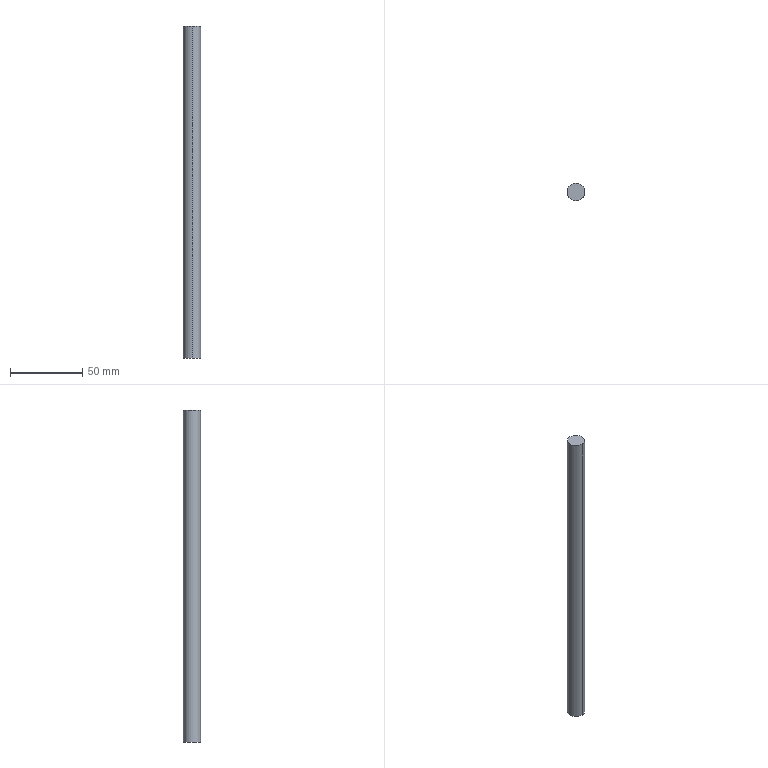Component | SolidWorks | Cylinder-1_TieRod-2 | 1 solid | 4 faces | box 12 x 12 x 230 mm | volume 26012 mm3 | cylinder 2 | plane 2 | commonest cylinder face diameters 12 x2
build123d program:
from build123d import *

# Parameters (mm, degrees)
SKETCH1_R           = 6
BOSS_EXTRUDE1_DEPTH = 230


with BuildPart() as part:
    # Sketch1 → Boss-Extrude1 (new body)
    with BuildSketch(Plane.XY):
        Circle(SKETCH1_R)
    extrude(amount=-BOSS_EXTRUDE1_DEPTH)


solid = part.part

# Placed as in the assembly
solid = solid.moved(Location((-152.557, 54.412, -158.451), (0, 0, 0)))
STEP:
#1=COLOUR_RGB('',0.7922,0.8196,0.9333);
#2=FILL_AREA_STYLE_COLOUR('',#1);
#3=FILL_AREA_STYLE('',(#2));
#4=SURFACE_STYLE_FILL_AREA(#3);
#5=SURFACE_SIDE_STYLE('',(#4));
#6=SURFACE_STYLE_USAGE(.BOTH.,#5);
#7=PRESENTATION_STYLE_ASSIGNMENT((#6));
#8=CARTESIAN_POINT('',(-6.006,1.906,-6.238));
#9=VERTEX_POINT('',#8);
#10=CARTESIAN_POINT('',(-6.006,2.378,-6.238));
#11=VERTEX_POINT('',#10);
#12=CARTESIAN_POINT('',(-6.006,2.142,-6.238));
#13=DIRECTION('',(0.,-0.,-1.));
#14=DIRECTION('',(0.,-1.,0.));
#15=AXIS2_PLACEMENT_3D('',#12,#13,#14);
#16=CIRCLE('',#15,0.2362);
#17=EDGE_CURVE('',#9,#11,#16,.T.);
#18=ORIENTED_EDGE('',*,*,#17,.T.);
#19=CARTESIAN_POINT('',(-6.006,2.378,-15.293));
#20=VERTEX_POINT('',#19);
#21=CARTESIAN_POINT('',(-6.006,2.378,-6.238));
#22=DIRECTION('',(0.,-0.,-1.));
#23=VECTOR('',#22,39.37);
#24=LINE('',#21,#23);
#25=EDGE_CURVE('',#11,#20,#24,.T.);
#26=ORIENTED_EDGE('',*,*,#25,.T.);
#27=CARTESIAN_POINT('',(-6.006,1.906,-15.293));
#28=VERTEX_POINT('',#27);
#29=CARTESIAN_POINT('',(-6.006,2.142,-15.293));
#30=DIRECTION('',(0.,-0.,-1.));
#31=DIRECTION('',(0.,-1.,0.));
#32=AXIS2_PLACEMENT_3D('',#29,#30,#31);
#33=CIRCLE('',#32,0.2362);
#34=EDGE_CURVE('',#28,#20,#33,.T.);
#35=ORIENTED_EDGE('',*,*,#34,.F.);
#36=CARTESIAN_POINT('',(-6.006,1.906,-6.238));
#37=DIRECTION('',(0.,-0.,-1.));
#38=VECTOR('',#37,39.37);
#39=LINE('',#36,#38);
#40=EDGE_CURVE('',#9,#28,#39,.T.);
#41=ORIENTED_EDGE('',*,*,#40,.F.);
#42=EDGE_LOOP('',(#18,#26,#35,#41));
#43=FACE_OUTER_BOUND('',#42,.T.);
#44=CARTESIAN_POINT('',(-6.006,2.142,-6.238));
#45=DIRECTION('',(0.,-0.,-1.));
#46=DIRECTION('',(0.,-1.,0.));
#47=AXIS2_PLACEMENT_3D('',#44,#45,#46);
#48=CYLINDRICAL_SURFACE('',#47,0.2362);
#49=ADVANCED_FACE('',(#43),#48,.T.);
#50=ORIENTED_EDGE('',*,*,#25,.F.);
#51=CARTESIAN_POINT('',(-6.006,2.142,-6.238));
#52=DIRECTION('',(0.,-0.,-1.));
#53=DIRECTION('',(0.,-1.,0.));
#54=AXIS2_PLACEMENT_3D('',#51,#52,#53);
#55=CIRCLE('',#54,0.2362);
#56=EDGE_CURVE('',#11,#9,#55,.T.);
#57=ORIENTED_EDGE('',*,*,#56,.T.);
#58=ORIENTED_EDGE('',*,*,#40,.T.);
#59=CARTESIAN_POINT('',(-6.006,2.142,-15.293));
#60=DIRECTION('',(0.,-0.,-1.));
#61=DIRECTION('',(0.,-1.,0.));
#62=AXIS2_PLACEMENT_3D('',#59,#60,#61);
#63=CIRCLE('',#62,0.2362);
#64=EDGE_CURVE('',#20,#28,#63,.T.);
#65=ORIENTED_EDGE('',*,*,#64,.F.);
#66=EDGE_LOOP('',(#50,#57,#58,#65));
#67=FACE_OUTER_BOUND('',#66,.T.);
#68=CARTESIAN_POINT('',(-6.006,2.142,-6.238));
#69=DIRECTION('',(0.,-0.,-1.));
#70=DIRECTION('',(0.,-1.,0.));
#71=AXIS2_PLACEMENT_3D('',#68,#69,#70);
#72=CYLINDRICAL_SURFACE('',#71,0.2362);
#73=ADVANCED_FACE('',(#67),#72,.T.);
#74=ORIENTED_EDGE('',*,*,#17,.F.);
#75=ORIENTED_EDGE('',*,*,#56,.F.);
#76=EDGE_LOOP('',(#74,#75));
#77=FACE_OUTER_BOUND('',#76,.T.);
#78=CARTESIAN_POINT('',(-6.006,2.142,-6.238));
#79=DIRECTION('',(0.,-0.,-1.));
#80=DIRECTION('',(-0.,-1.,0.));
#81=AXIS2_PLACEMENT_3D('',#78,#79,#80);
#82=PLANE('',#81);
#83=ADVANCED_FACE('',(#77),#82,.F.);
#84=ORIENTED_EDGE('',*,*,#34,.T.);
#85=ORIENTED_EDGE('',*,*,#64,.T.);
#86=EDGE_LOOP('',(#84,#85));
#87=FACE_OUTER_BOUND('',#86,.T.);
#88=CARTESIAN_POINT('',(-6.006,2.142,-15.293));
#89=DIRECTION('',(0.,-0.,-1.));
#90=DIRECTION('',(-0.,-1.,0.));
#91=AXIS2_PLACEMENT_3D('',#88,#89,#90);
#92=PLANE('',#91);
#93=ADVANCED_FACE('',(#87),#92,.T.);
#94=CLOSED_SHELL('',(#49,#73,#83,#93));
#95=MANIFOLD_SOLID_BREP('',#94);
#96=STYLED_ITEM('',(#7),#95);
#97=PRESENTATION_LAYER_ASSIGNMENT('','',(#96));
#98=CARTESIAN_POINT('',(0.,0.,0.));
#99=DIRECTION('',(0.,0.,1.));
#100=DIRECTION('',(1.,0.,0.));
#101=AXIS2_PLACEMENT_3D('',#98,#99,#100);
#102=(LENGTH_UNIT()NAMED_UNIT(*)SI_UNIT($,.METRE.));
#103=LENGTH_MEASURE_WITH_UNIT(LENGTH_MEASURE(0.0254),#102);
#104=DIMENSIONAL_EXPONENTS(1.,0.,0.,0.,0.,0.,0.);
#105=(CONVERSION_BASED_UNIT('',#103)LENGTH_UNIT()NAMED_UNIT(#104));
#106=UNCERTAINTY_MEASURE_WITH_UNIT(LENGTH_MEASURE(0.00001),#105,'','');
#107=(NAMED_UNIT(*)PLANE_ANGLE_UNIT()SI_UNIT($,.RADIAN.));
#108=(NAMED_UNIT(*)SI_UNIT($,.STERADIAN.)SOLID_ANGLE_UNIT());
#109=(GEOMETRIC_REPRESENTATION_CONTEXT(3)GLOBAL_UNCERTAINTY_ASSIGNED_CONTEXT((#106))GLOBAL_UNIT_ASSIGNED_CONTEXT((#105,#107,#108))REPRESENTATION_CONTEXT('',''));
#110=ADVANCED_BREP_SHAPE_REPRESENTATION('',(#95,#101),#109);
#111=(LENGTH_UNIT()NAMED_UNIT(*)SI_UNIT($,.METRE.));
#112=LENGTH_MEASURE_WITH_UNIT(LENGTH_MEASURE(0.0254),#111);
#113=DIMENSIONAL_EXPONENTS(1.,0.,0.,0.,0.,0.,0.);
#114=(CONVERSION_BASED_UNIT('',#112)LENGTH_UNIT()NAMED_UNIT(#113));
#115=UNCERTAINTY_MEASURE_WITH_UNIT(LENGTH_MEASURE(0.00001),#114,'','');
#116=(NAMED_UNIT(*)PLANE_ANGLE_UNIT()SI_UNIT($,.RADIAN.));
#117=(NAMED_UNIT(*)SI_UNIT($,.STERADIAN.)SOLID_ANGLE_UNIT());
#118=(GEOMETRIC_REPRESENTATION_CONTEXT(3)GLOBAL_UNCERTAINTY_ASSIGNED_CONTEXT((#115))GLOBAL_UNIT_ASSIGNED_CONTEXT((#114,#116,#117))REPRESENTATION_CONTEXT('',''));
#119=MECHANICAL_DESIGN_GEOMETRIC_PRESENTATION_REPRESENTATION('',(#96),#118);